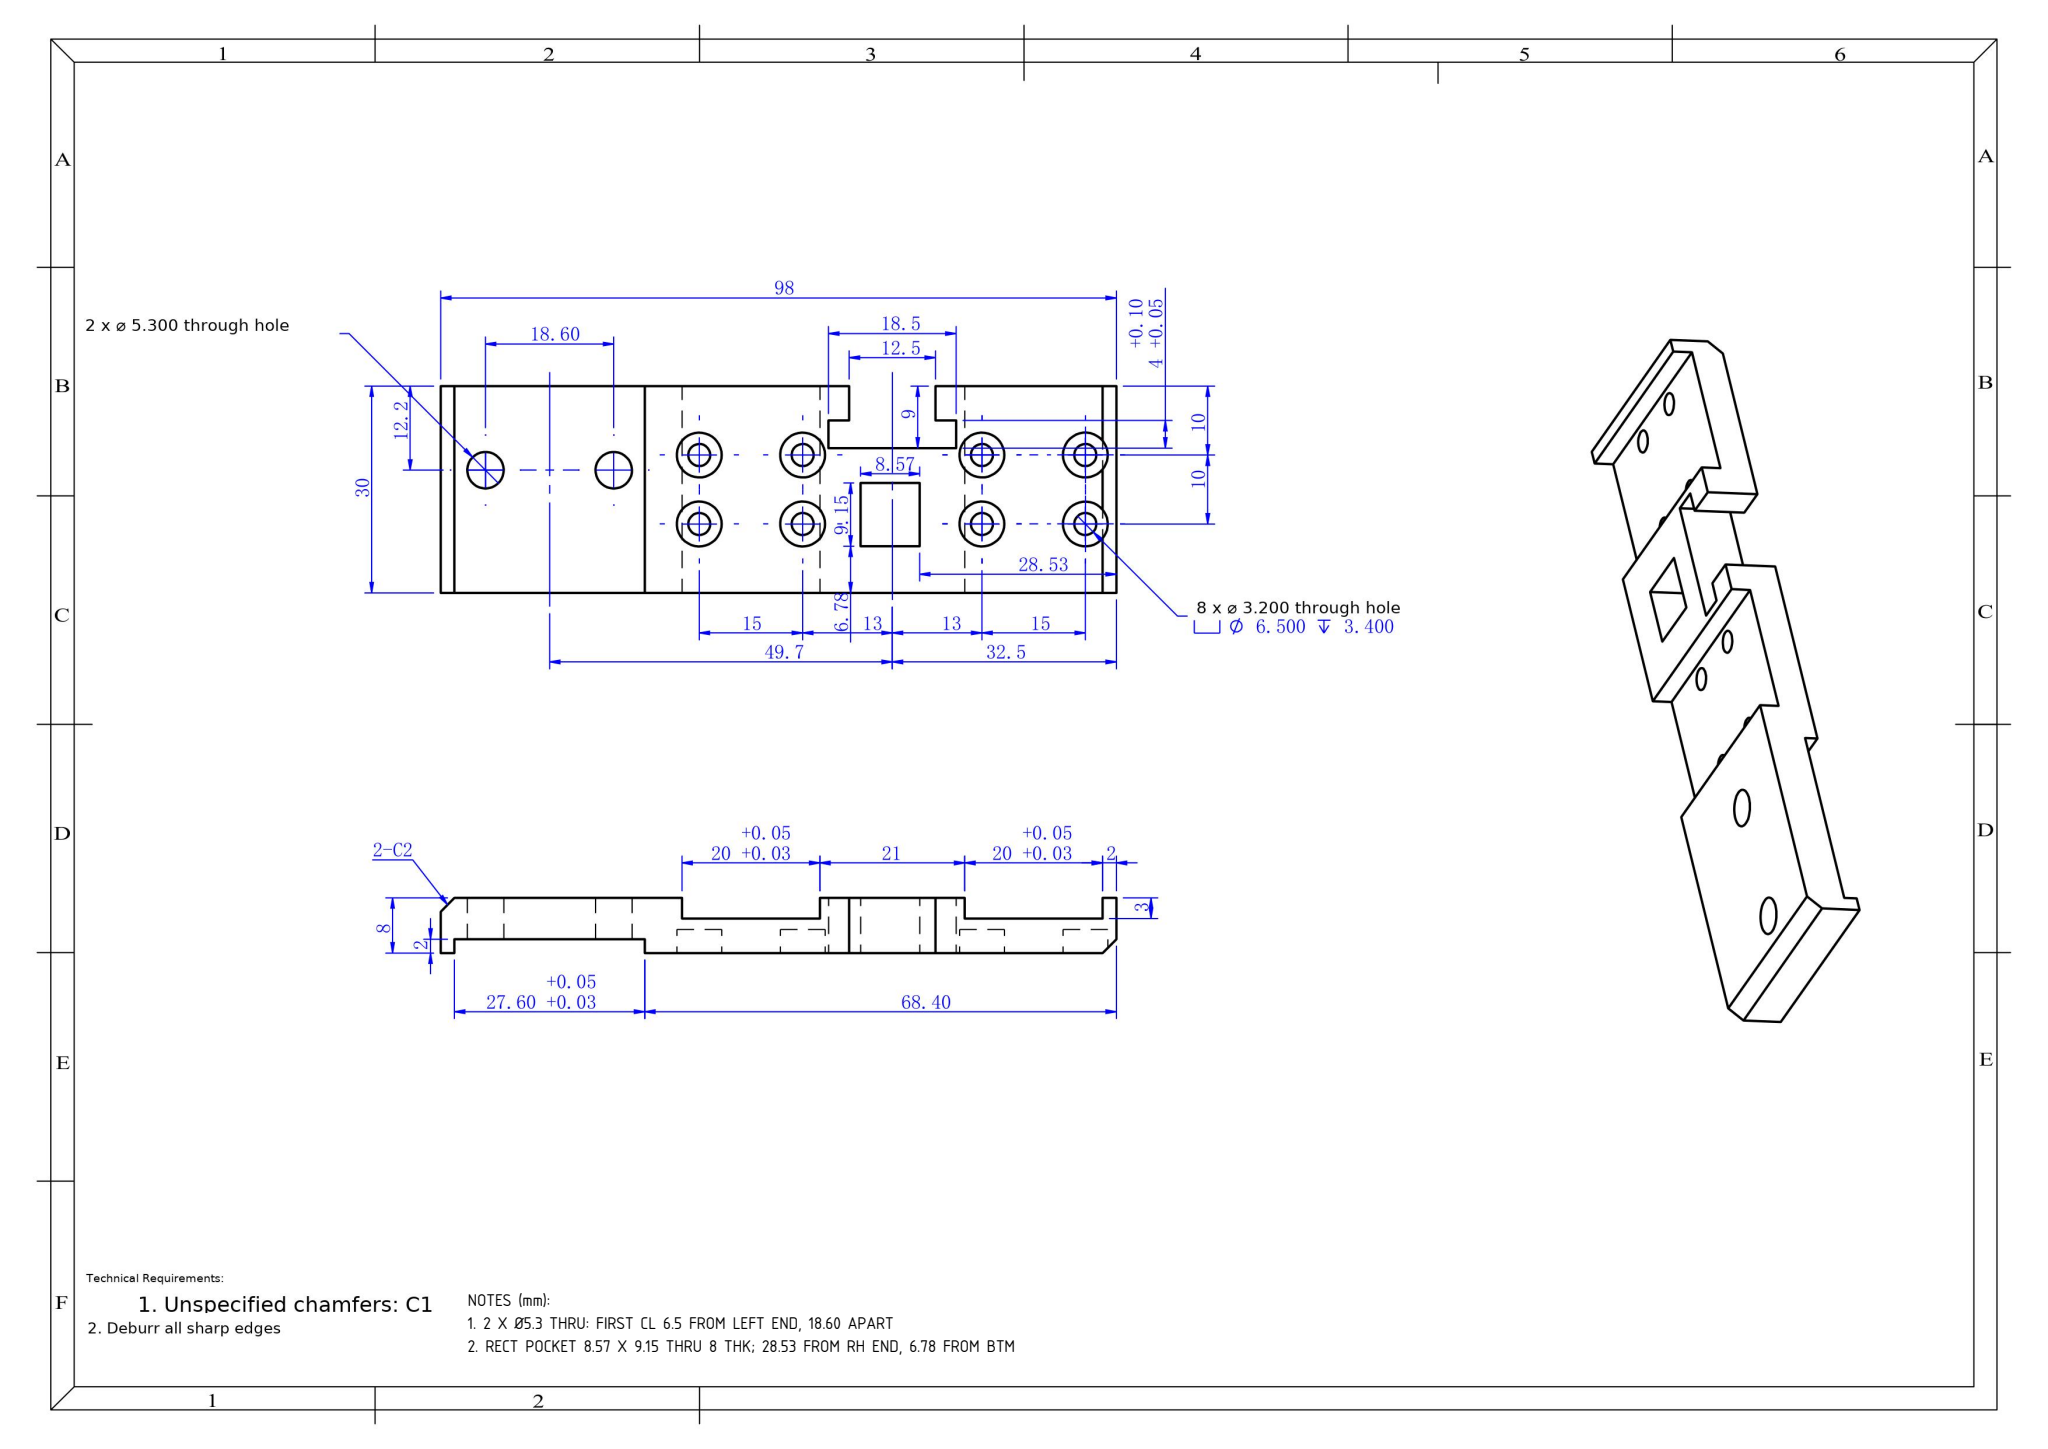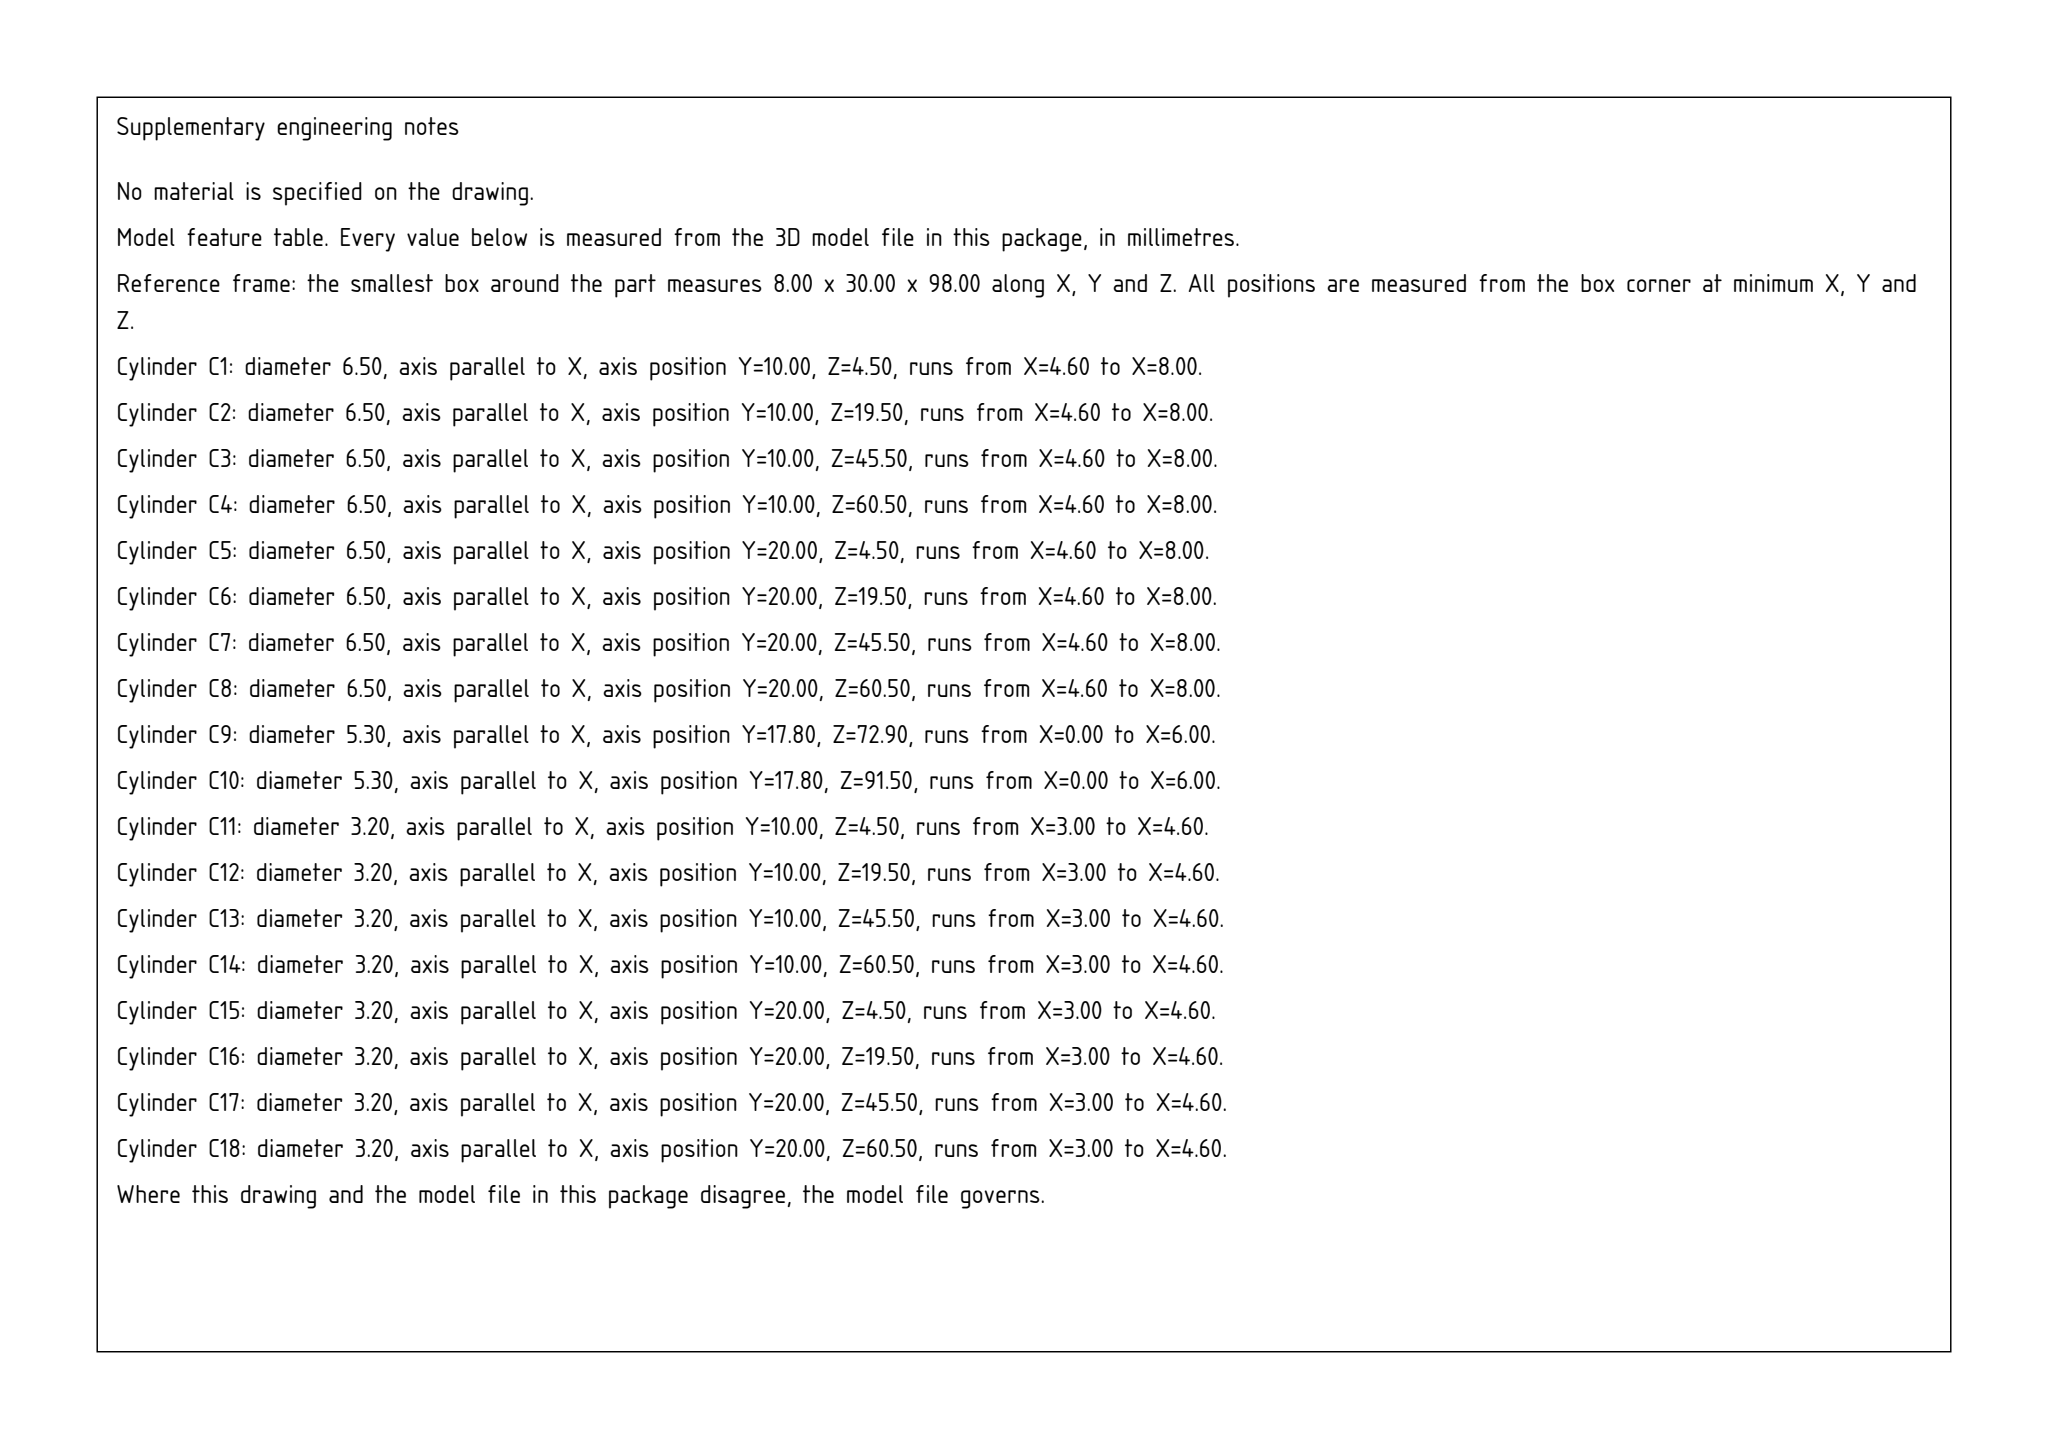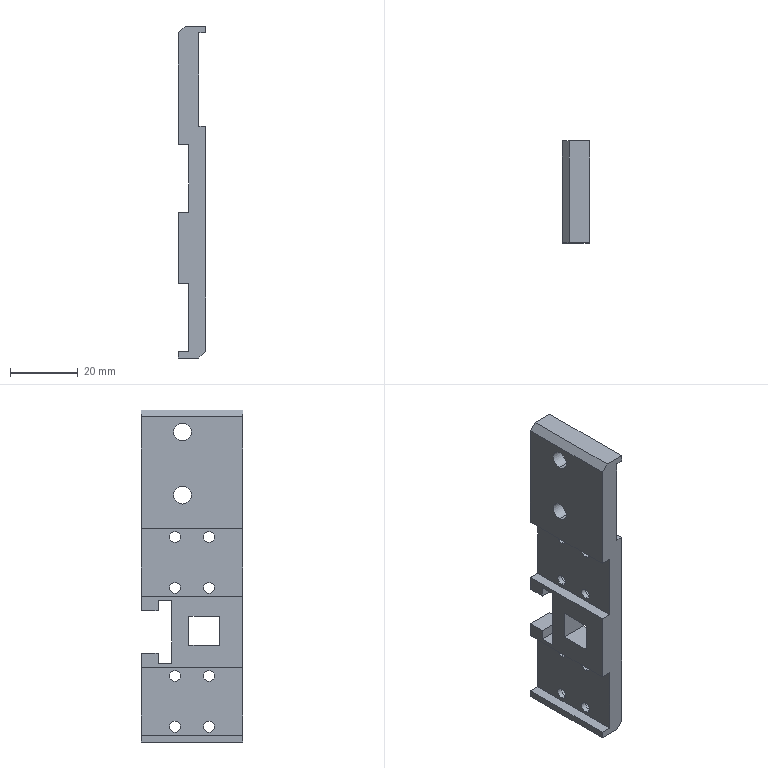Part | SolidWorks | mm | 1 solid | 76 faces | box 8 x 30 x 98 mm | volume 15156 mm3 | plane 40 | cylinder 36 | commonest cylinder face diameters 6.5 x16 3.2 x16 5.3 x4
Drawing notes:
2 X Ø5.3 THRU: FIRST CL 6.5 FROM LEFT END, 18.60 APART | from the solid: Ø5.3 cylinders at z=91.5 & 72.9; part z length 98 -> 98-91.5=6.5, spacing 18.6
RECT POCKET 8.57 X 9.15 THRU 8 THK; 28.53 FROM RH END, 6.78 FROM BTM | from the solid: z planes 28.53 & 37.10 (8.57), y planes 6.78 & 15.93 (9.15); no bottom face -> thru 8 thk
build123d program:
from build123d import *

# Parameters (mm, degrees)
SKETCH1_W                                       = 8
SKETCH1_H                                       = 30
BOSS_EXTRUDE1_DEPTH                             = 98
SKETCH2_W                                       = 3
SKETCH2_H                                       = 20
CUT_EXTRUDE1_DEPTH                              = 125.052
CUT_EXTRUDE2_DEPTH                              = 106.308
SKETCH7_W                                       = 2
SKETCH7_H                                       = 27.6
CUT_EXTRUDE4_DEPTH                              = 125.052
CHAMFER1_SIZE                                   = 2
CHAMFER2_SIZE                                   = 2
M3_HEX_SOCKET_HEAD_CAP_SCREW_CBORE1_D           = 3.2
M3_HEX_SOCKET_HEAD_CAP_SCREW_CBORE1_CBORE_D     = 6.5
M3_HEX_SOCKET_HEAD_CAP_SCREW_CBORE1_CBORE_DEPTH = 3.4
F_5_3_5_3_DIAMETER_HOLE1_D                      = 5.3
SKETCH13_W                                      = 8.569
SKETCH13_H                                      = 9.147
CUT_EXTRUDE5_DEPTH                              = 10


with BuildPart() as part:
    # Sketch1 → Boss-Extrude1 (new body)
    with BuildSketch(Plane.XY):
        with Locations((65.893, -22.708)):
            Rectangle(SKETCH1_W, SKETCH1_H)
    extrude(amount=BOSS_EXTRUDE1_DEPTH)

    # Sketch2 → Cut-Extrude1 (cut, through all)
    with BuildSketch(Plane(origin=(0, -7.708, 0), x_dir=(1, 0, 0), z_dir=(0, 1, 0))):
        with Locations((63.393, -53)):
            Rectangle(SKETCH2_W, SKETCH2_H)
        with Locations((63.393, -12)):
            Rectangle(SKETCH2_W, SKETCH2_H)
    extrude(amount=-CUT_EXTRUDE1_DEPTH, mode=Mode.SUBTRACT)

    # Sketch5 → Cut-Extrude2 (cut, through all)
    with BuildSketch(Plane.ZY.offset(-61.893)):
        Polygon((23.25, -12.708), (26.25, -12.708), (26.25, -7.708), (38.75, -7.708), (38.75, -12.708), (41.75, -12.708), (41.75, -16.708), (23.25, -16.708), align=None)
    extrude(amount=-CUT_EXTRUDE2_DEPTH, mode=Mode.SUBTRACT)

    # Sketch7 → Cut-Extrude4 (cut, through all)
    with BuildSketch(Plane(origin=(0, -7.708, 0), x_dir=(1, 0, 0), z_dir=(0, 1, 0))):
        with Locations((68.893, -82.2)):
            Rectangle(SKETCH7_W, SKETCH7_H)
    extrude(amount=-CUT_EXTRUDE4_DEPTH, mode=Mode.SUBTRACT)

    # Chamfer1
    chamfer1_edges = [part.edges().sort_by_distance(p)[0] for p in [
        (61.893, -22.708, 98),
    ]]
    chamfer(chamfer1_edges, length=CHAMFER1_SIZE)

    # Chamfer2
    chamfer2_edges = [part.edges().sort_by_distance(p)[0] for p in [
        (69.893, -22.708, 0),
    ]]
    chamfer(chamfer2_edges, length=CHAMFER2_SIZE)

    # M3 Hex Socket Head Cap Screw CBORE1 (through all)
    with Locations(Plane(origin=(69.893, 0, 0), x_dir=(0, 0, -1), z_dir=(1, 0, 0))):
        with Locations((-60.5, -17.708), (-45.5, -17.708), (-45.5, -27.708), (-60.5, -27.708), (-19.5, -17.708), (-19.5, -27.708), (-4.5, -17.708), (-4.5, -27.708)):
            CounterBoreHole(M3_HEX_SOCKET_HEAD_CAP_SCREW_CBORE1_D / 2, M3_HEX_SOCKET_HEAD_CAP_SCREW_CBORE1_CBORE_D / 2, M3_HEX_SOCKET_HEAD_CAP_SCREW_CBORE1_CBORE_DEPTH)

    # 5.3 _5.3_ Diameter Hole1 (through all)
    with Locations(Plane.ZY.offset(-61.893)):
        with Locations((72.9, -19.908), (91.5, -19.908)):
            Hole(F_5_3_5_3_DIAMETER_HOLE1_D / 2)

    # Sketch13 → Cut-Extrude5 (cut)
    with BuildSketch(Plane.ZY.offset(-61.893)):
        with Locations((32.814, -26.351)):
            Rectangle(SKETCH13_W, SKETCH13_H)
    extrude(amount=-CUT_EXTRUDE5_DEPTH, mode=Mode.SUBTRACT)


solid = part.part